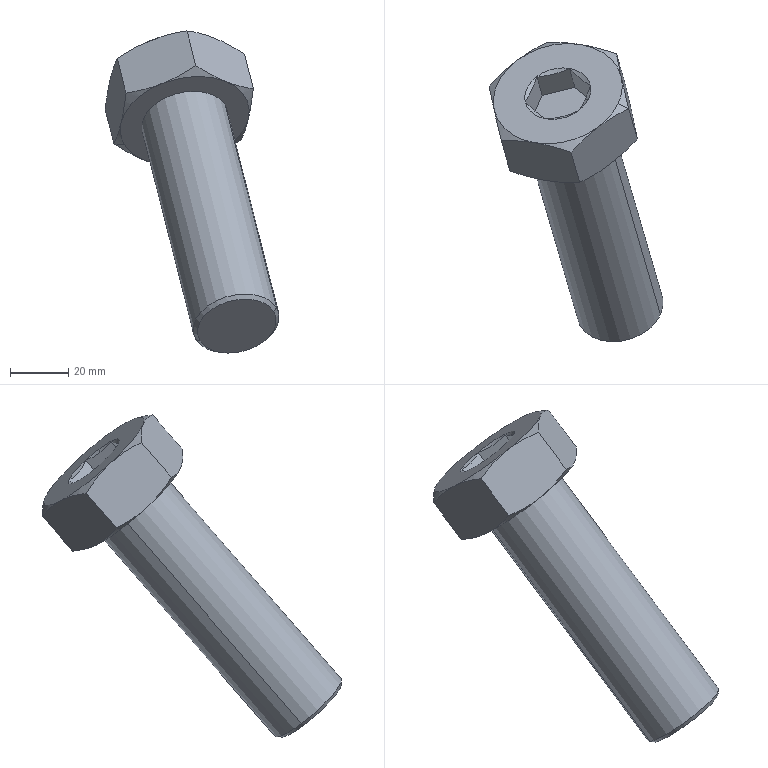Component | SolidWorks | Bolt15x65-2 | 1 solid | 41 faces | volume 98466 mm3 | cone 23 | plane 16 | cylinder 2 | commonest cylinder face diameters 30 x2 | material Ti-3Al-8V-6Cr-4Mo-4Zr (SS)